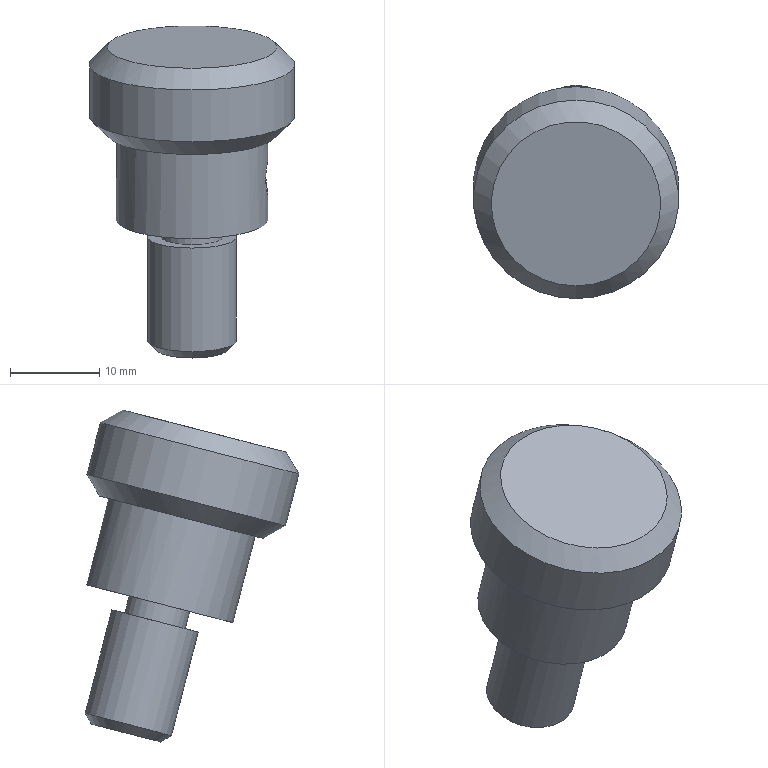Component | NX | TONGQISAI | 1 solid | 14 faces | volume 7130 mm3 | plane 6 | cylinder 5 | cone 3 | commonest cylinder face diameters 17 x1 23 x1 7 x1 10 x1 4 x1